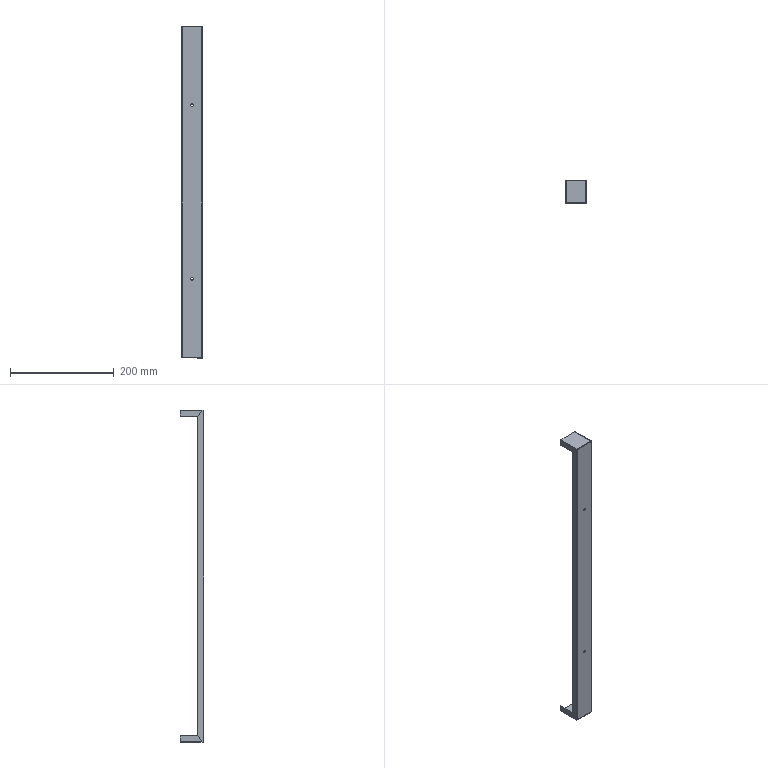Component | SolidWorks | CabinetWelding-1_TopLightBracket-1 | 1 solid | 82 faces | volume 44160 mm3 | plane 54 | cylinder 20 | spline 8 | commonest cylinder face diameters 2.2 x7 0.2 x7 5 x4 2.4 x1 0.4 x1